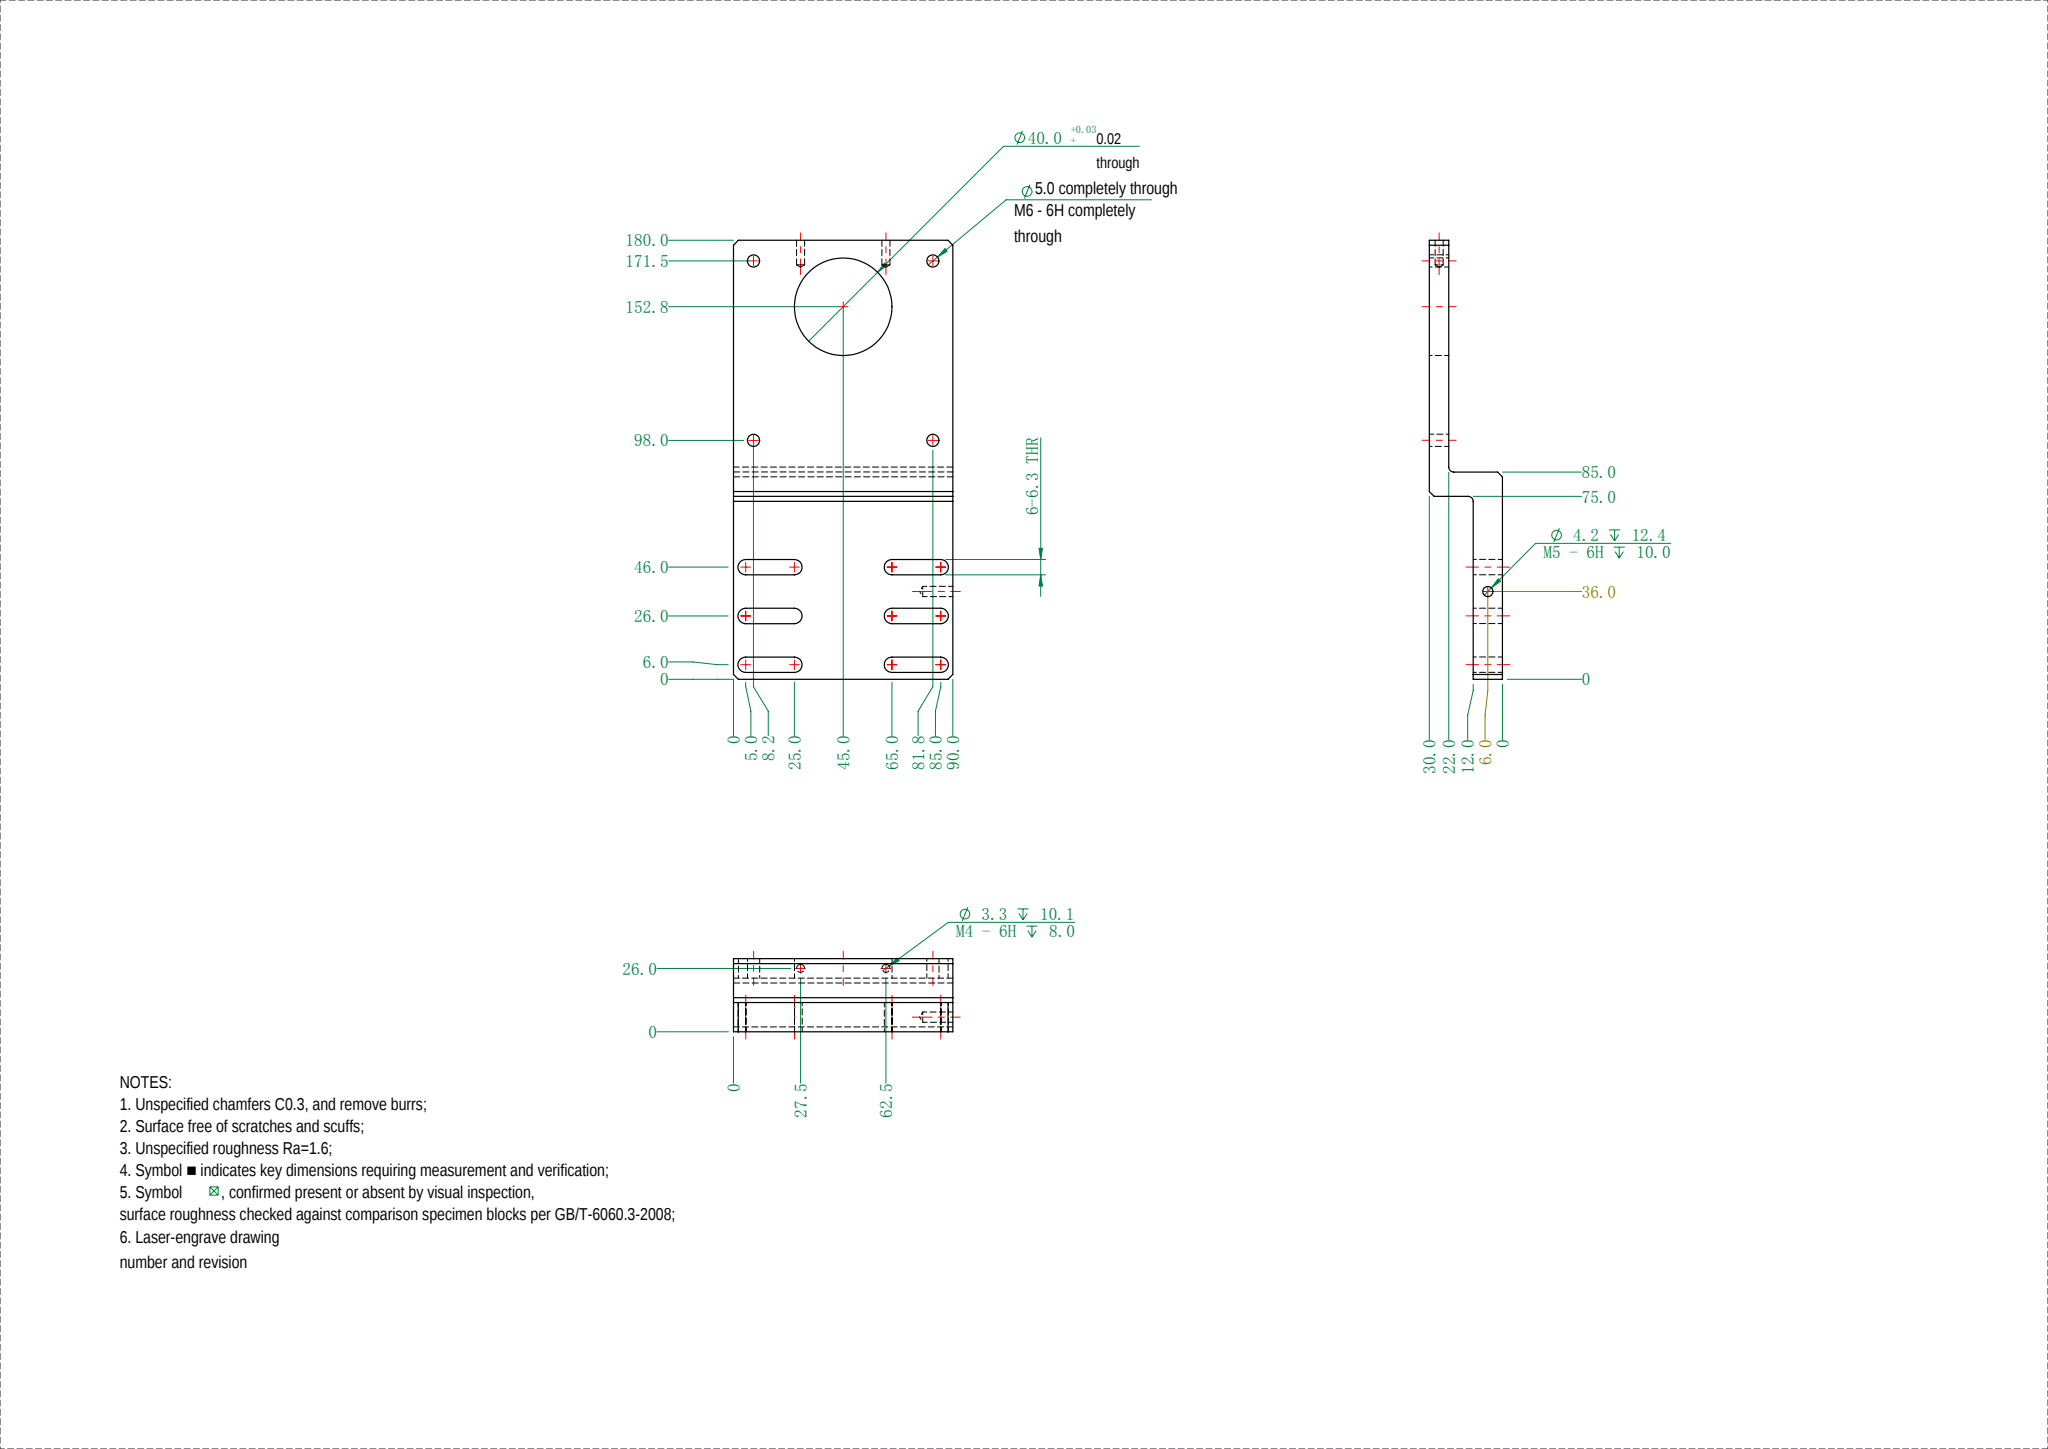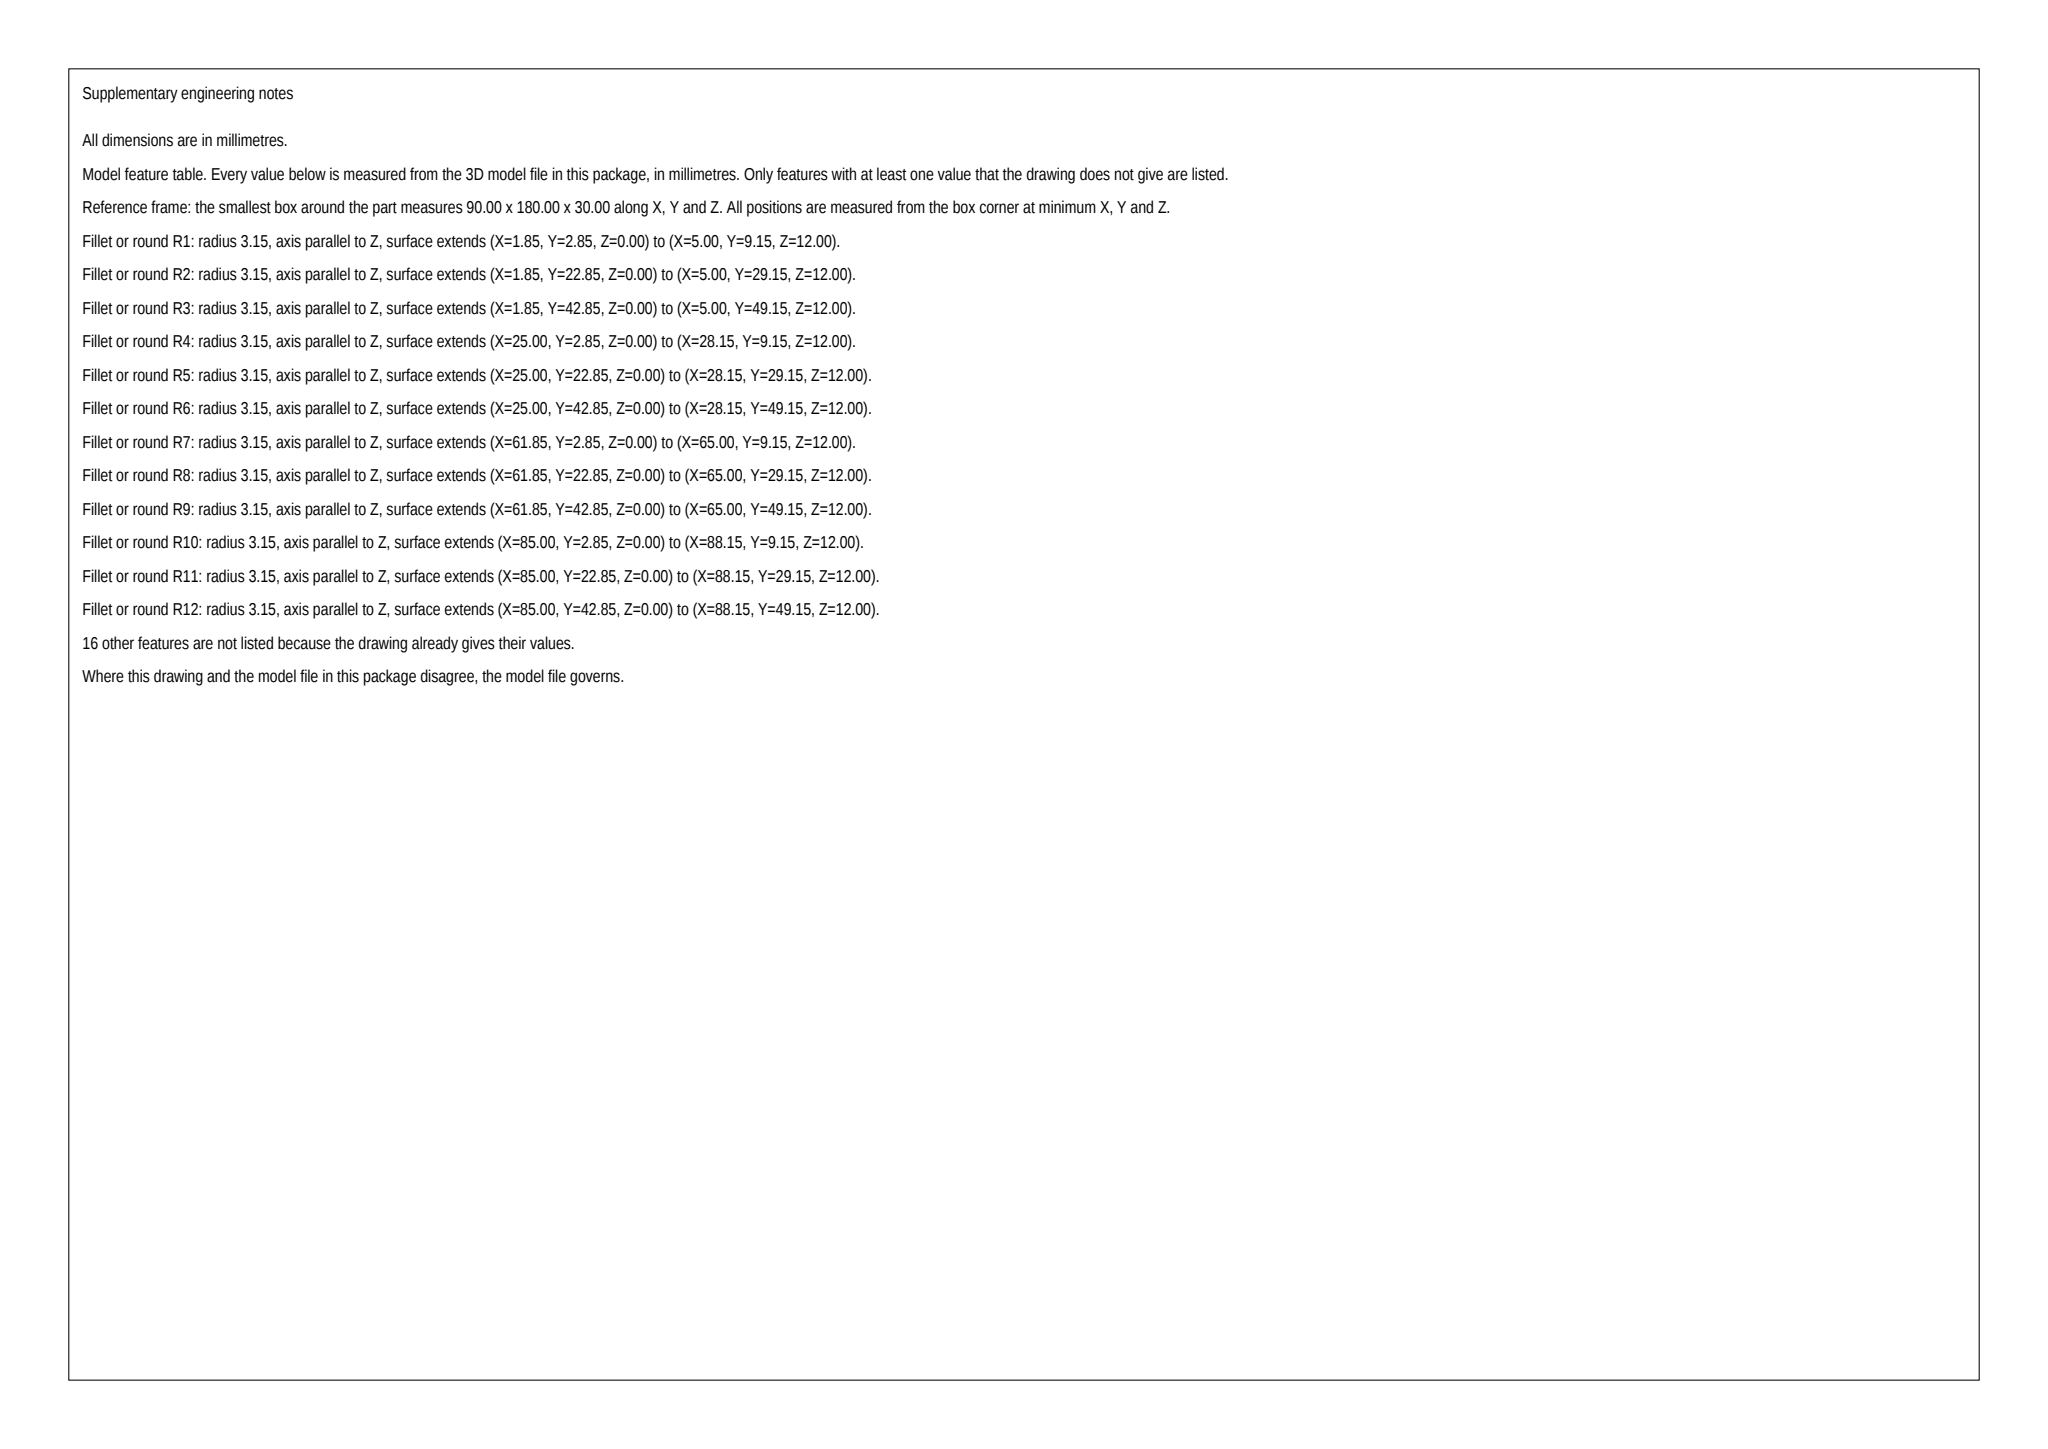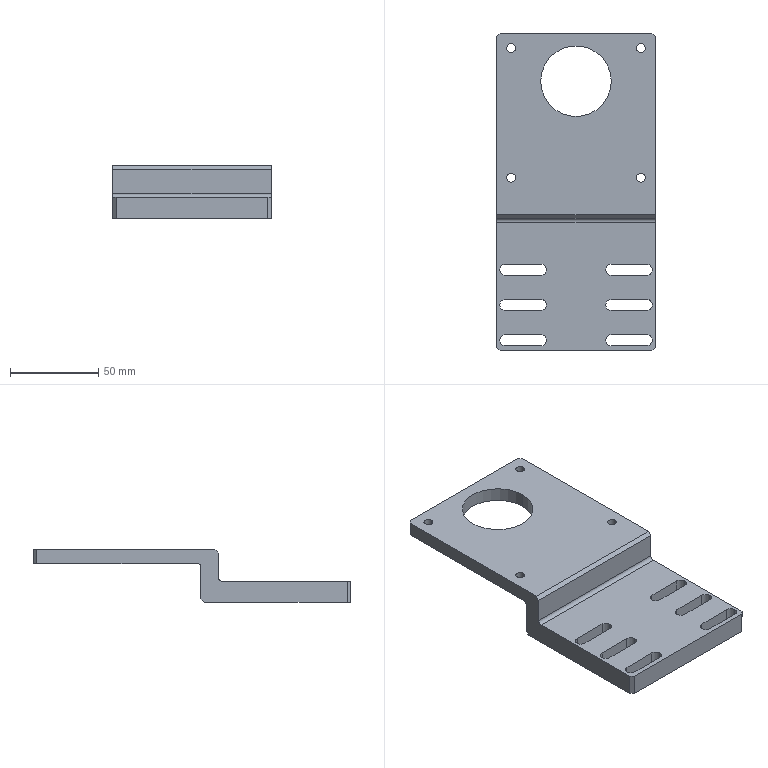Part | SolidWorks | mm | 1 solid | 70 faces | box 90 x 180 x 30 mm | volume 153761 mm3 | cylinder 36 | plane 28 | cone 6 | commonest cylinder face diameters 6.3 x18 5 x8 3.3 x4 4.2 x2 40 x2 4 x2
Drawing notes:
6 SLOTS 6.3 WIDE x 26.3 LG (20.0 C-C), R3.15 ENDS, THRU 12 | from the solid: Ø6.3 z-axis cyls L=12 paired x=5/25 & 65/85 at y=6/26/46; plate z 0-12
2X M4-6H (BOTTOM): X 27.5 & 62.5 FROM LEFT EDGE, 26.0 FROM BASE | from the solid: Ø3.3 y-axis cyls at [27.5,-,26.0] & [62.5,-,26.0], L=10.1, csk cone 118°
2X M5-6H (SIDE): 36.0 FROM Y0, 6.0 FROM Z0 BOTTOM FACE | from the solid: Ø4.2 x-axis cyls at [-,36.0,6.0], L=12.4, qty 2, cone 118°
Ø4.0 THRU 90 WIDTH, 73.0 FROM BTM, 14.0 FROM BACK FACE | from the solid: cylinder dia 4.0 axis x, pos [null,73.0,14.0], length 90.0 (full bbox X)
Ø4.0 THRU 90 WIDTH, 87.0 FROM BTM, 20.0 FROM BACK FACE | from the solid: cylinder dia 4.0 axis x, pos [null,87.0,20.0], length 90.0 (full bbox X)
build123d program:
from build123d import *

# Parameters (mm, degrees)
SKETCH1_W             = 90
SKETCH1_H             = 180
EXTRUDE1_DEPTH        = 30
M6_TAPPED_HOLE1_D     = 5
SKETCH4_R             = 20
CUT_EXTRUDE1_DEPTH    = 106
CUT_EXTRUDE1_2_DEPTH  = 106
SKETCH2_2_W           = 90
SKETCH2_2_H           = 95
CUT_EXTRUDE2_DEPTH    = 22
SKETCH3_2_W           = 90
SKETCH3_2_H           = 75
CUT_EXTRUDE3_DEPTH    = 18
M4_TAPPED_HOLE1_D     = 3.3
M4_TAPPED_HOLE1_DEPTH = 10.1
M4_TAPPED_HOLE1_TIP   = 0.9914
CHAMFER1_SIZE         = 2
FILLET1_R             = 2
LPATTERN1_COUNT       = 3
LPATTERN1_PITCH       = 20
M5_TAPPED_HOLE1_D     = 4.2
M5_TAPPED_HOLE1_DEPTH = 12.4
M5_TAPPED_HOLE1_TIP   = 1.262


with BuildPart() as part:
    # Sketch1 → Extrude1 (new body)
    with BuildSketch(Plane.XY):
        Rectangle(SKETCH1_W, SKETCH1_H)
    extrude(amount=EXTRUDE1_DEPTH)

    # M6 Tapped Hole1 (through all)
    with Locations(Plane.XY.offset(30)):
        with Locations((-36.77, 81.52), (-36.77, 7.98), (36.77, 81.52), (36.77, 7.98)):
            Hole(M6_TAPPED_HOLE1_D / 2)

    # Sketch4 → Cut-Extrude1 (cut, through all)
    with BuildSketch(Plane.XY.offset(30)):
        with Locations((0, 62.75)):
            Circle(SKETCH4_R)
    extrude(amount=-CUT_EXTRUDE1_DEPTH, mode=Mode.SUBTRACT)

    # Sketch1_2 → Cut-Extrude1_2 (cut, through all)
    with BuildSketch(Plane.XY.offset(30)):
        with BuildLine():
            Line((-40, -80.85), (-20, -80.85))
            ThreePointArc((-20, -80.85), (-16.85, -84), (-20, -87.15))
            Line((-20, -87.15), (-40, -87.15))
            ThreePointArc((-40, -87.15), (-43.15, -84), (-40, -80.85))
        make_face()
        with BuildLine():
            Line((20, -80.85), (40, -80.85))
            ThreePointArc((40, -80.85), (43.15, -84), (40, -87.15))
            Line((40, -87.15), (20, -87.15))
            ThreePointArc((20, -87.15), (16.85, -84), (20, -80.85))
        make_face()
    cut_extrude1_2 = extrude(amount=-CUT_EXTRUDE1_2_DEPTH, mode=Mode.SUBTRACT)

    # Sketch2_2 → Cut-Extrude2 (cut)
    with BuildSketch(Plane(origin=(0, 0, 0), x_dir=(-1, 0, 0), z_dir=(0, 0, -1))):
        with Locations((0, 42.5)):
            Rectangle(SKETCH2_2_W, SKETCH2_2_H)
    extrude(amount=-CUT_EXTRUDE2_DEPTH, mode=Mode.SUBTRACT)

    # Sketch3_2 → Cut-Extrude3 (cut)
    with BuildSketch(Plane.XY.offset(30)):
        with Locations((0, -52.5)):
            Rectangle(SKETCH3_2_W, SKETCH3_2_H)
    extrude(amount=-CUT_EXTRUDE3_DEPTH, mode=Mode.SUBTRACT)

    # M4 Tapped Hole1
    with Locations(Plane(origin=(0, 90, 0), x_dir=(1, 0, 0), z_dir=(0, 1, 0))):
        with Locations((-17.5, -26), (17.5, -26)):
            Hole(M4_TAPPED_HOLE1_D / 2, depth=M4_TAPPED_HOLE1_DEPTH)
            with Locations((0, 0, -(M4_TAPPED_HOLE1_DEPTH + M4_TAPPED_HOLE1_TIP / 2))):  # 118° drill point
                Cone(0, M4_TAPPED_HOLE1_D / 2, M4_TAPPED_HOLE1_TIP, mode=Mode.SUBTRACT)

    # Chamfer1
    chamfer1_edges = [part.edges().sort_by_distance(p)[0] for p in [
        (45, -90, 6),
        (-45, -90, 6),
        (0, -15, 30),
        (0, -5, 0),
        (-45, 90, 26),
        (45, 90, 26),
    ]]
    chamfer(chamfer1_edges, length=CHAMFER1_SIZE)

    # Fillet1
    fillet1_edges = [part.edges().sort_by_distance(p)[0] for p in [
        (0, -15, 12),
        (0, -5, 22),
    ]]
    fillet(fillet1_edges, radius=FILLET1_R)

    # LPattern1: Cut-Extrude1_2 ×3
    with Locations(*[(0, i * LPATTERN1_PITCH, 0) for i in range(1, LPATTERN1_COUNT)]):
        add(cut_extrude1_2, mode=Mode.SUBTRACT)

    # M5 Tapped Hole1
    with Locations(Plane(origin=(45, 0, 0), x_dir=(0, 0, -1), z_dir=(1, 0, 0))):
        with Locations((-6, -54)):
            Hole(M5_TAPPED_HOLE1_D / 2, depth=M5_TAPPED_HOLE1_DEPTH)
            with Locations((0, 0, -(M5_TAPPED_HOLE1_DEPTH + M5_TAPPED_HOLE1_TIP / 2))):  # 118° drill point
                Cone(0, M5_TAPPED_HOLE1_D / 2, M5_TAPPED_HOLE1_TIP, mode=Mode.SUBTRACT)


solid = part.part